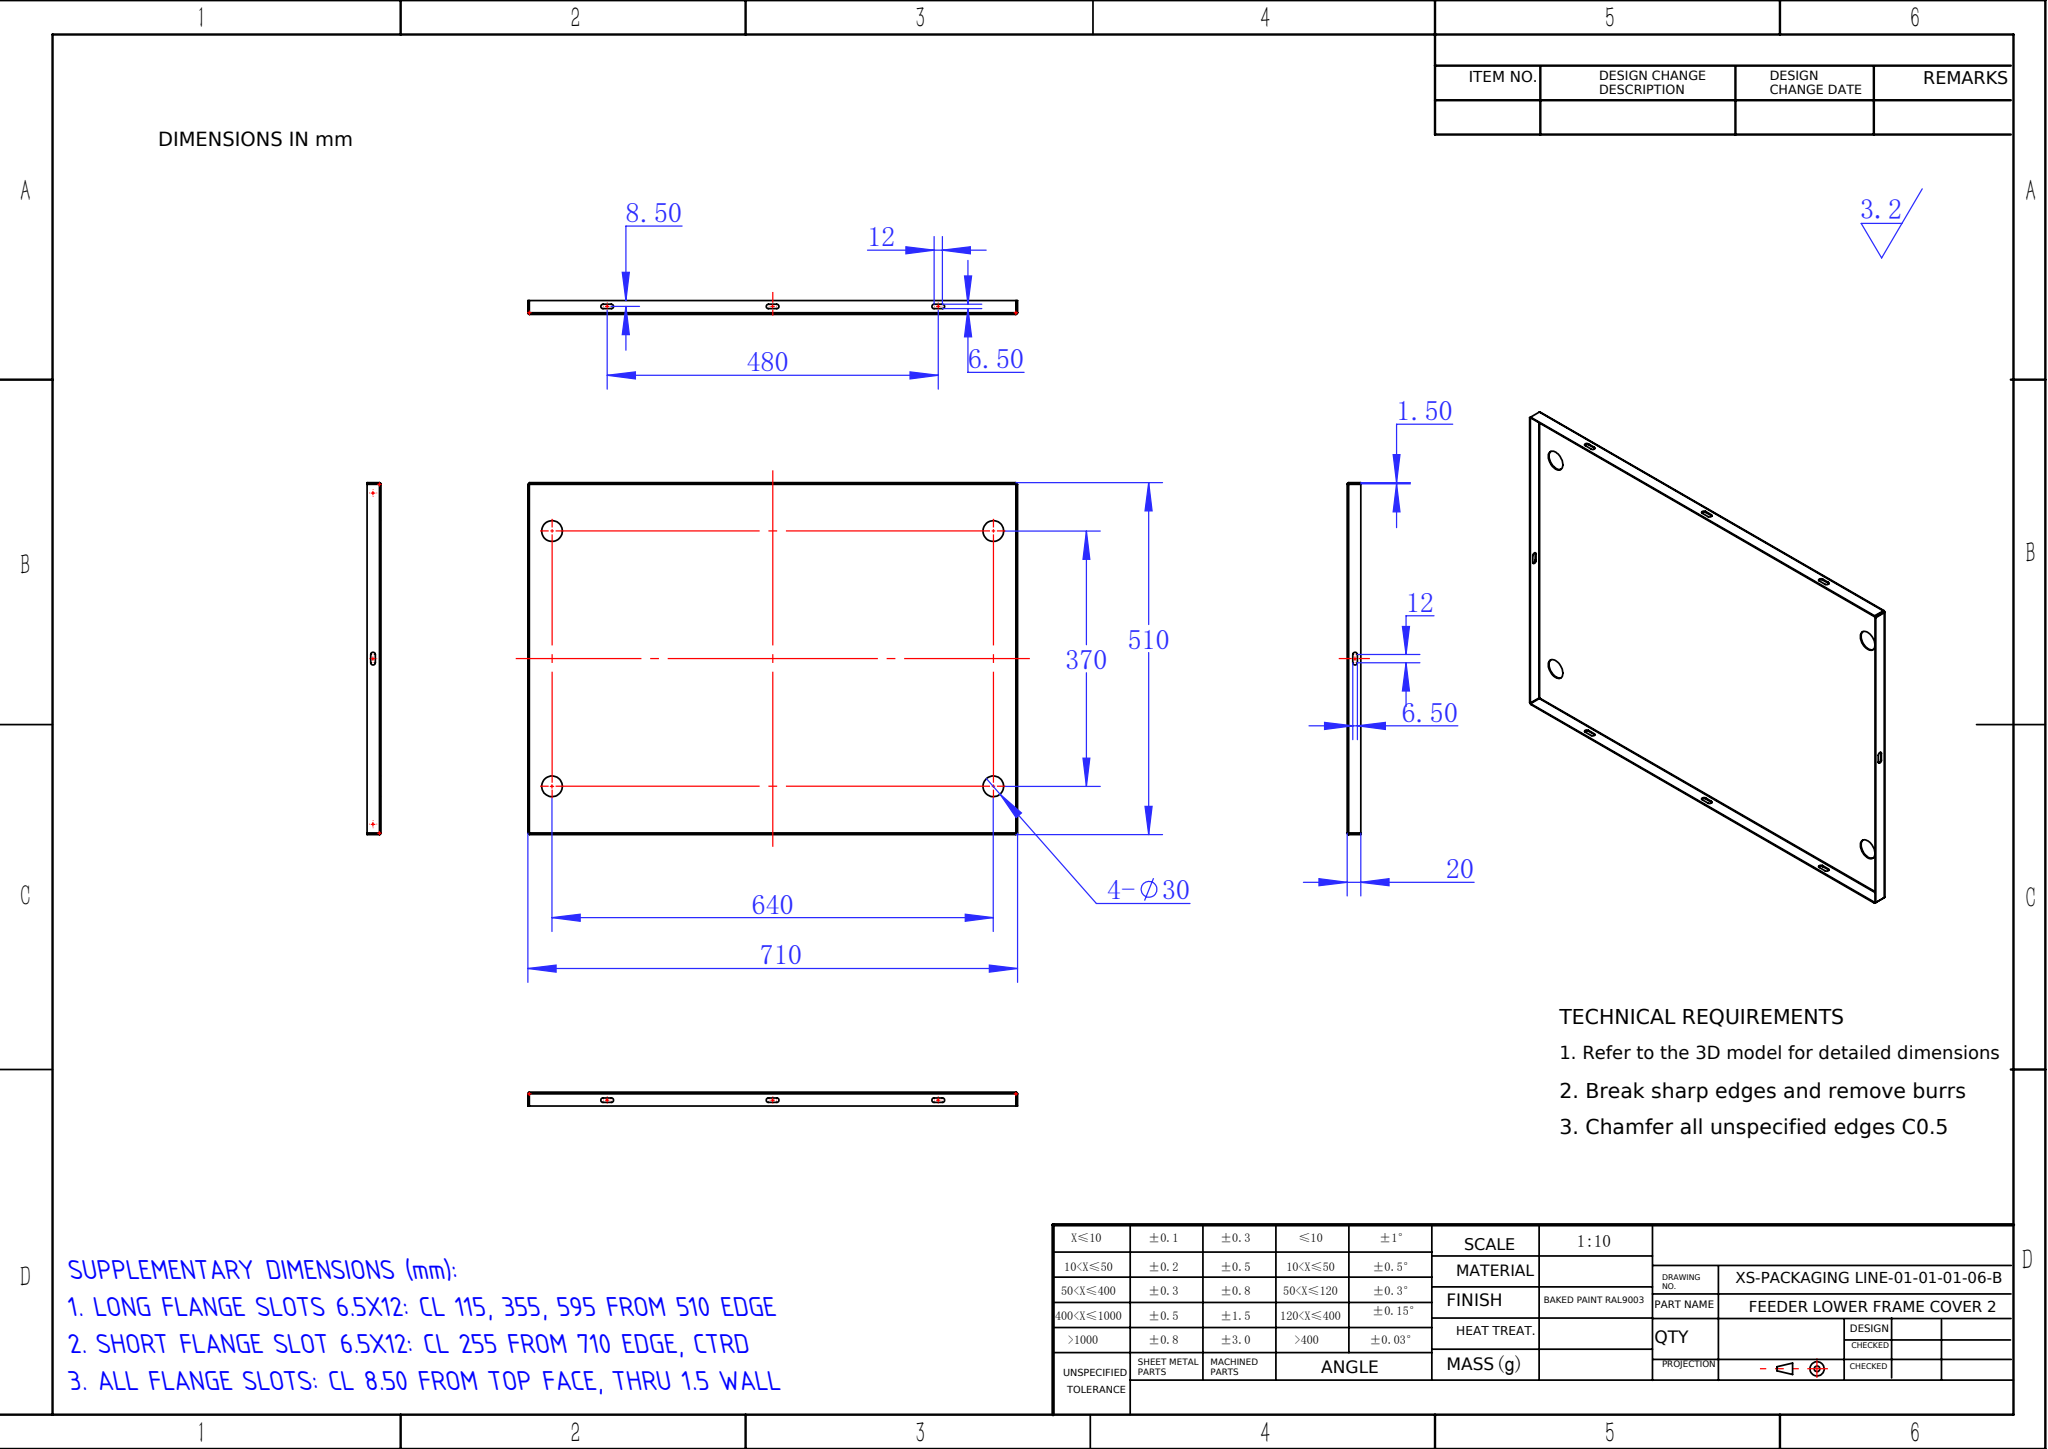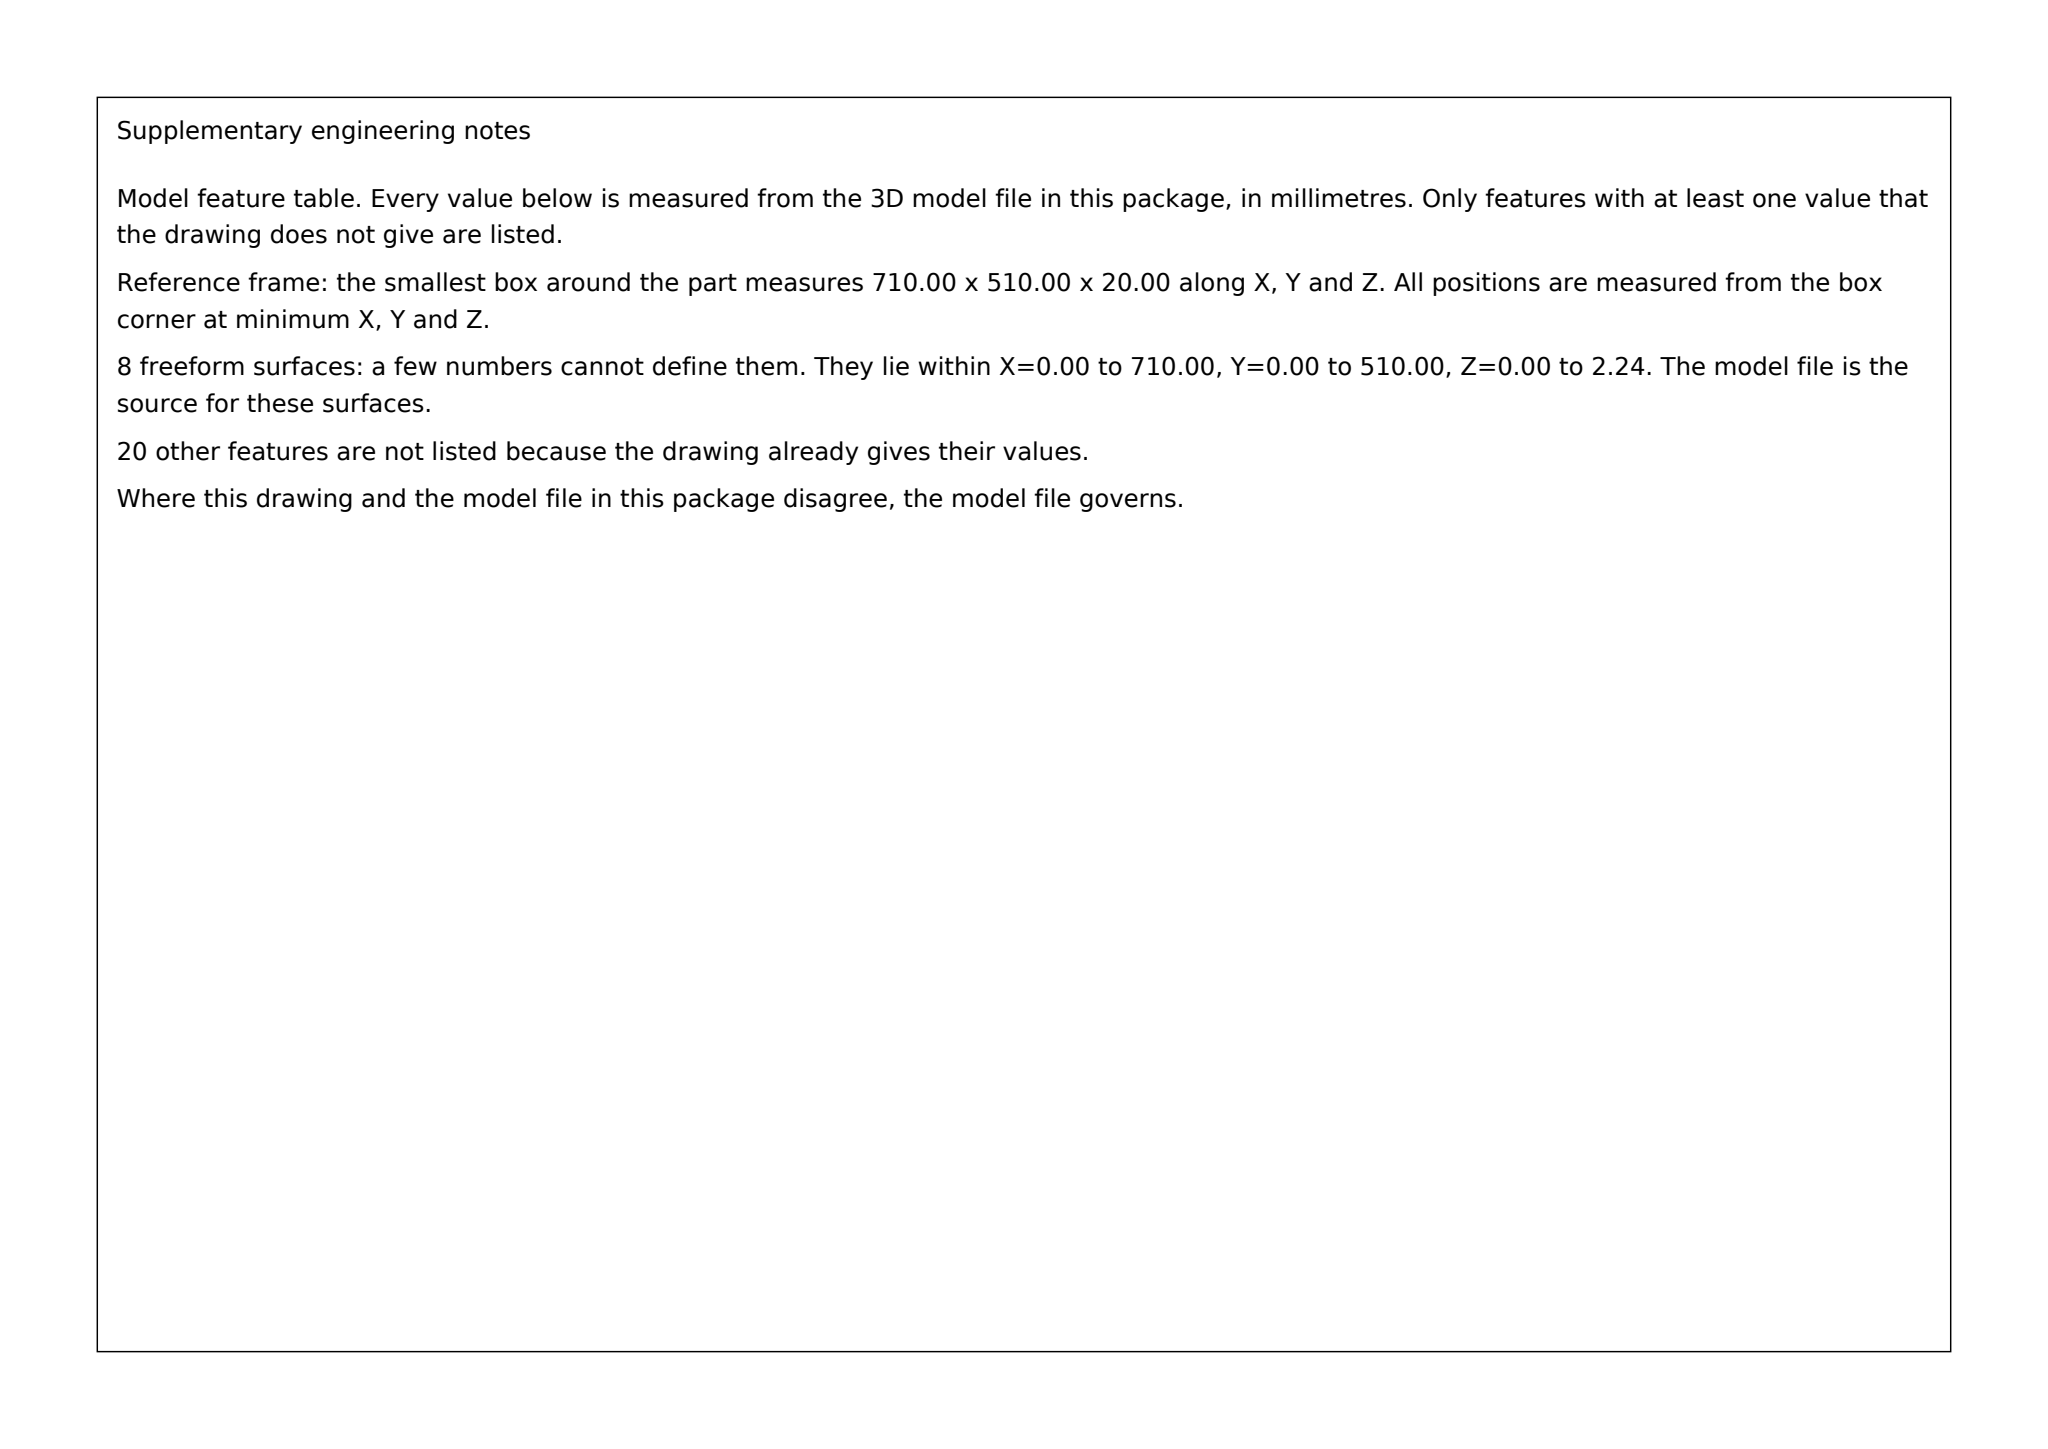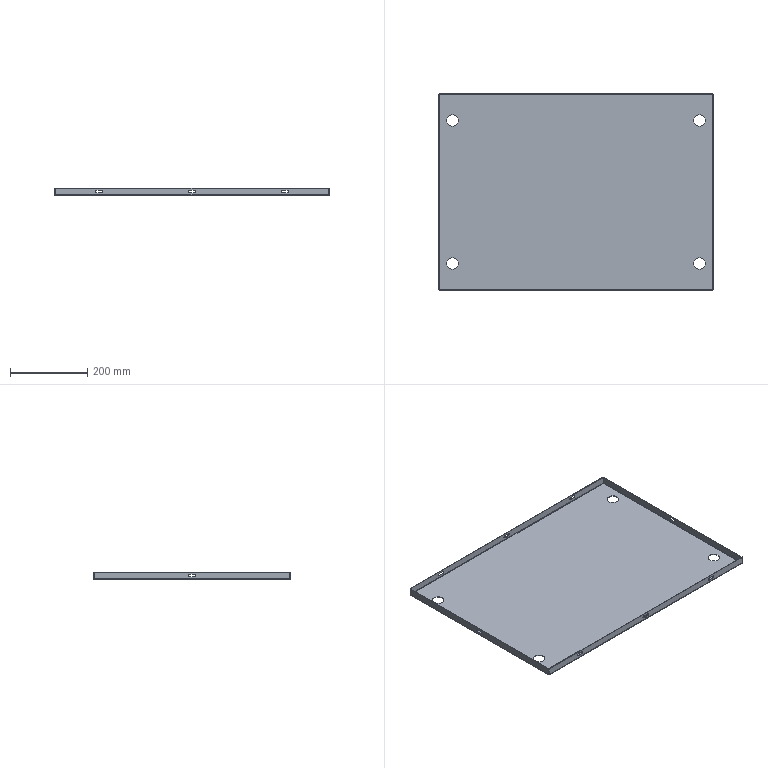Part | SolidWorks | mm | 1 solid | 78 faces | box 710 x 510 x 20 mm | volume 602447 mm3 | plane 38 | cylinder 32 | spline 8 | commonest cylinder face diameters 6.5 x16 30 x8 4.473 x4 1.473 x4